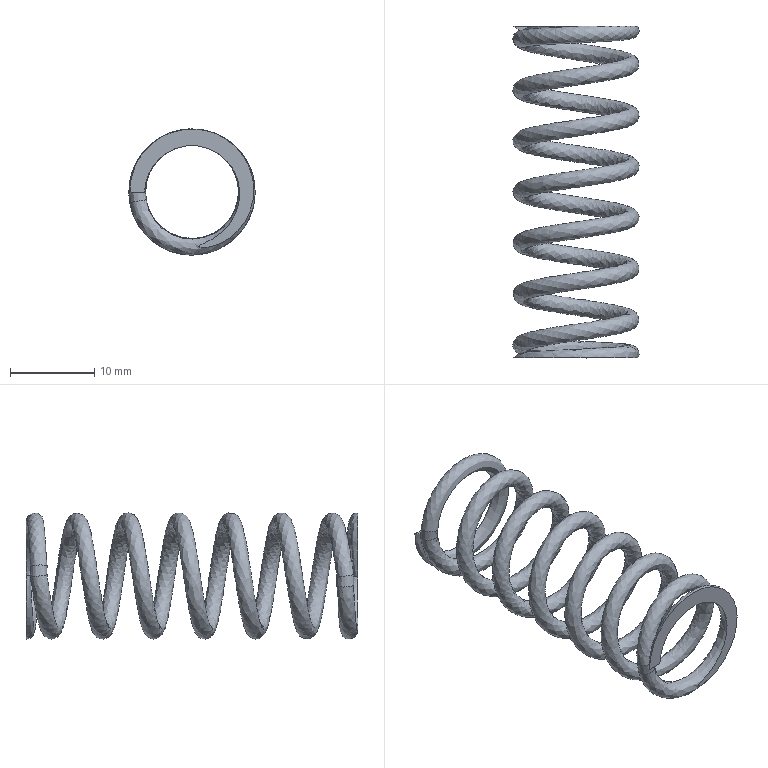Component | NX | VENT_SPRING | 1 solid | 9 faces | volume 945 mm3 | spline 5 | plane 4